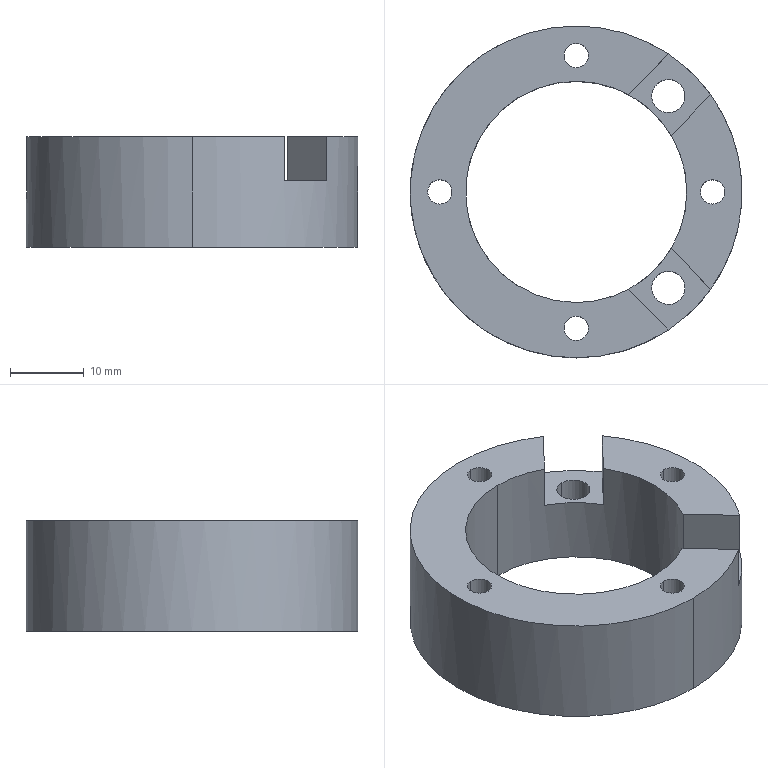CAM job | Mastercam | mm | 4 operations | part box 45 x 45 x 15
1. Contour (Ramp) | 6 - 6 平铣刀
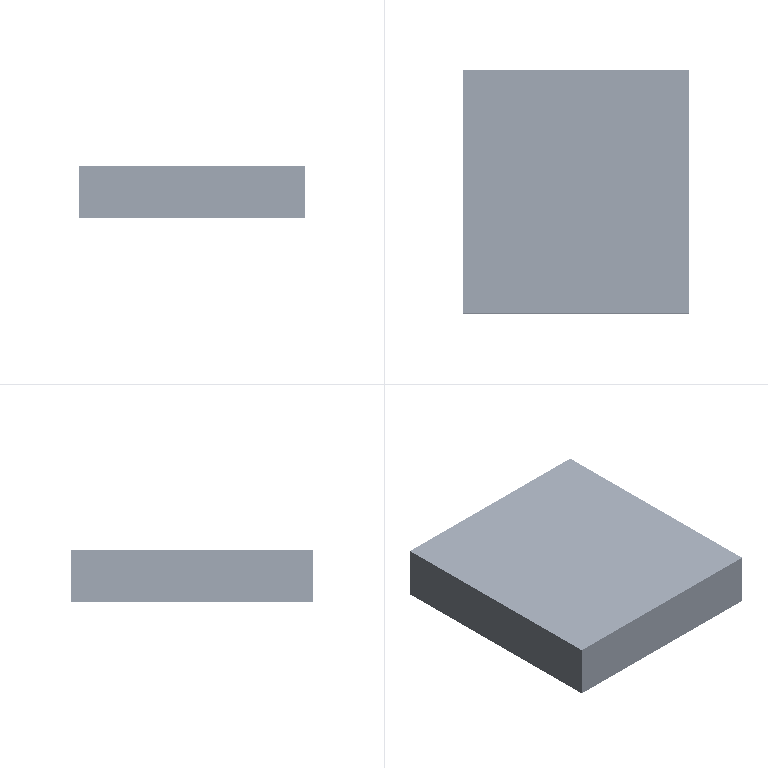2. Contour (2D) | 6 - 6 平铣刀
3. Drill/Counterbore | 7 - 4 倒角刀
4. Contour (2D chamfer) | 7 - 4 倒角刀